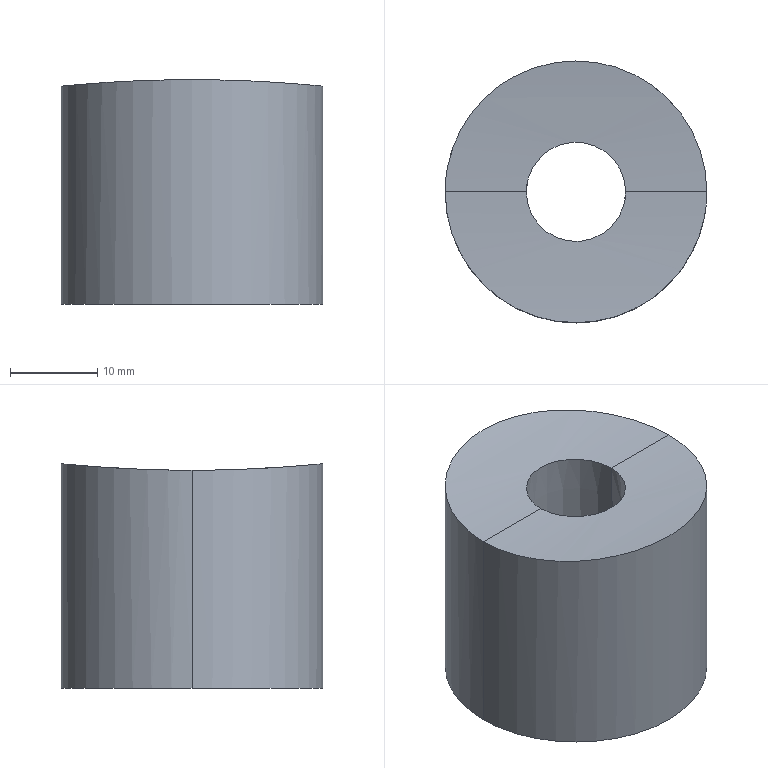Component | SolidWorks | JF21-80.1-1-3(_)-1-SOLID13-1 | 1 solid | 7 faces | box 30 x 30 x 25.75 mm | volume 14893 mm3 | cylinder 4 | cone 2 | plane 1 | commonest cylinder face diameters 300 x2 30 x2
STEP:
#1=COLOUR_RGB('',0.7922,0.8196,0.9333);
#2=FILL_AREA_STYLE_COLOUR('',#1);
#3=FILL_AREA_STYLE('',(#2));
#4=SURFACE_STYLE_FILL_AREA(#3);
#5=SURFACE_SIDE_STYLE('',(#4));
#6=SURFACE_STYLE_USAGE(.BOTH.,#5);
#7=PRESENTATION_STYLE_ASSIGNMENT((#6));
#8=CARTESIAN_POINT('',(10.8,-39.37,30.315));
#9=VERTEX_POINT('',#8);
#10=CARTESIAN_POINT('',(11.248,-39.37,30.315));
#11=VERTEX_POINT('',#10);
#12=CARTESIAN_POINT('',(10.8,-39.37,30.315));
#13=CARTESIAN_POINT('',(10.8,-39.385,30.315));
#14=CARTESIAN_POINT('',(10.801,-39.399,30.315));
#15=CARTESIAN_POINT('',(10.805,-39.421,30.315));
#16=CARTESIAN_POINT('',(10.807,-39.428,30.315));
#17=CARTESIAN_POINT('',(10.811,-39.442,30.315));
#18=CARTESIAN_POINT('',(10.814,-39.449,30.315));
#19=CARTESIAN_POINT('',(10.822,-39.469,30.316));
#20=CARTESIAN_POINT('',(10.829,-39.482,30.316));
#21=CARTESIAN_POINT('',(10.845,-39.507,30.317));
#22=CARTESIAN_POINT('',(10.855,-39.518,30.317));
#23=CARTESIAN_POINT('',(10.876,-39.539,30.317));
#24=CARTESIAN_POINT('',(10.887,-39.548,30.318));
#25=CARTESIAN_POINT('',(10.905,-39.56,30.318));
#26=CARTESIAN_POINT('',(10.912,-39.564,30.318));
#27=CARTESIAN_POINT('',(10.924,-39.571,30.318));
#28=CARTESIAN_POINT('',(10.931,-39.574,30.318));
#29=CARTESIAN_POINT('',(10.951,-39.583,30.319));
#30=CARTESIAN_POINT('',(10.965,-39.587,30.319));
#31=CARTESIAN_POINT('',(10.994,-39.593,30.319));
#32=CARTESIAN_POINT('',(11.009,-39.594,30.319));
#33=CARTESIAN_POINT('',(11.038,-39.594,30.319));
#34=CARTESIAN_POINT('',(11.053,-39.593,30.319));
#35=CARTESIAN_POINT('',(11.082,-39.587,30.319));
#36=CARTESIAN_POINT('',(11.096,-39.583,30.319));
#37=CARTESIAN_POINT('',(11.116,-39.574,30.318));
#38=CARTESIAN_POINT('',(11.123,-39.571,30.318));
#39=CARTESIAN_POINT('',(11.136,-39.564,30.318));
#40=CARTESIAN_POINT('',(11.142,-39.56,30.318));
#41=CARTESIAN_POINT('',(11.16,-39.548,30.318));
#42=CARTESIAN_POINT('',(11.171,-39.539,30.317));
#43=CARTESIAN_POINT('',(11.192,-39.518,30.317));
#44=CARTESIAN_POINT('',(11.202,-39.507,30.317));
#45=CARTESIAN_POINT('',(11.214,-39.489,30.316));
#46=CARTESIAN_POINT('',(11.218,-39.482,30.316));
#47=CARTESIAN_POINT('',(11.225,-39.469,30.316));
#48=CARTESIAN_POINT('',(11.228,-39.463,30.316));
#49=CARTESIAN_POINT('',(11.236,-39.442,30.315));
#50=CARTESIAN_POINT('',(11.24,-39.428,30.315));
#51=CARTESIAN_POINT('',(11.246,-39.4,30.315));
#52=CARTESIAN_POINT('',(11.248,-39.385,30.315));
#53=CARTESIAN_POINT('',(11.248,-39.37,30.315));
#54=B_SPLINE_CURVE_WITH_KNOTS('',3,(#12,#13,#14,#15,#16,#17,#18,#19,#20,#21,#22,#23,#24,#25,#26,#27,#28,#29,#30,#31,#32,#33,#34,#35,#36,#37,#38,#39,#40,#41,#42,#43,#44,#45,#46,#47,#48,#49,#50,#51,#52,#53),.UNSPECIFIED.,.F.,.F.,(4,2,2,2,2,2,2,2,2,2,2,2,2,2,2,2,2,2,2,2,4),(0.,0.001112,0.001667,0.002223,0.003335,0.004447,0.005558,0.006114,0.00667,0.007782,0.008893,0.01,0.01112,0.01167,0.01223,0.01334,0.01445,0.01501,0.01556,0.01667,0.01779),.UNSPECIFIED.);
#55=EDGE_CURVE('',#9,#11,#54,.T.);
#56=ORIENTED_EDGE('',*,*,#55,.T.);
#57=CARTESIAN_POINT('',(11.278,-39.37,29.331));
#58=VERTEX_POINT('',#57);
#59=CARTESIAN_POINT('',(11.278,-39.37,29.331));
#60=DIRECTION('',(-0.0312,-0.,0.9995));
#61=VECTOR('',#60,39.37);
#62=LINE('',#59,#61);
#63=EDGE_CURVE('',#58,#11,#62,.T.);
#64=ORIENTED_EDGE('',*,*,#63,.F.);
#65=CARTESIAN_POINT('',(10.769,-39.37,29.331));
#66=VERTEX_POINT('',#65);
#67=CARTESIAN_POINT('',(11.024,-39.37,29.331));
#68=DIRECTION('',(0.,0.,-1.));
#69=DIRECTION('',(-1.,0.,0.));
#70=AXIS2_PLACEMENT_3D('',#67,#68,#69);
#71=CIRCLE('',#70,0.2548);
#72=EDGE_CURVE('',#58,#66,#71,.T.);
#73=ORIENTED_EDGE('',*,*,#72,.T.);
#74=CARTESIAN_POINT('',(10.769,-39.37,29.331));
#75=DIRECTION('',(0.0312,0.,0.9995));
#76=VECTOR('',#75,39.37);
#77=LINE('',#74,#76);
#78=EDGE_CURVE('',#66,#9,#77,.T.);
#79=ORIENTED_EDGE('',*,*,#78,.T.);
#80=EDGE_LOOP('',(#56,#64,#73,#79));
#81=FACE_OUTER_BOUND('',#80,.T.);
#82=CARTESIAN_POINT('',(11.024,-39.37,29.331));
#83=DIRECTION('',(0.,0.,-1.));
#84=DIRECTION('',(1.,0.,0.));
#85=AXIS2_PLACEMENT_3D('',#82,#83,#84);
#86=CONICAL_SURFACE('',#85,0.2548,0.03121);
#87=ADVANCED_FACE('',(#81),#86,.F.);
#88=CARTESIAN_POINT('',(11.614,-39.37,30.315));
#89=VERTEX_POINT('',#88);
#90=CARTESIAN_POINT('',(10.433,-39.37,30.315));
#91=VERTEX_POINT('',#90);
#92=CARTESIAN_POINT('',(11.614,-39.37,30.315));
#93=CARTESIAN_POINT('',(11.614,-39.331,30.315));
#94=CARTESIAN_POINT('',(11.61,-39.293,30.315));
#95=CARTESIAN_POINT('',(11.599,-39.236,30.316));
#96=CARTESIAN_POINT('',(11.594,-39.217,30.317));
#97=CARTESIAN_POINT('',(11.583,-39.18,30.318));
#98=CARTESIAN_POINT('',(11.577,-39.162,30.319));
#99=CARTESIAN_POINT('',(11.554,-39.108,30.321));
#100=CARTESIAN_POINT('',(11.536,-39.074,30.322));
#101=CARTESIAN_POINT('',(11.504,-39.026,30.325));
#102=CARTESIAN_POINT('',(11.492,-39.01,30.326));
#103=CARTESIAN_POINT('',(11.468,-38.98,30.328));
#104=CARTESIAN_POINT('',(11.455,-38.966,30.329));
#105=CARTESIAN_POINT('',(11.414,-38.925,30.332));
#106=CARTESIAN_POINT('',(11.384,-38.901,30.334));
#107=CARTESIAN_POINT('',(11.336,-38.868,30.336));
#108=CARTESIAN_POINT('',(11.319,-38.858,30.337));
#109=CARTESIAN_POINT('',(11.285,-38.84,30.339));
#110=CARTESIAN_POINT('',(11.25,-38.824,30.34));
#111=CARTESIAN_POINT('',(11.214,-38.811,30.342));
#112=CARTESIAN_POINT('',(11.177,-38.799,30.343));
#113=CARTESIAN_POINT('',(11.158,-38.795,30.343));
#114=CARTESIAN_POINT('',(11.101,-38.783,30.344));
#115=CARTESIAN_POINT('',(11.063,-38.78,30.345));
#116=CARTESIAN_POINT('',(11.005,-38.78,30.345));
#117=CARTESIAN_POINT('',(10.985,-38.78,30.344));
#118=CARTESIAN_POINT('',(10.947,-38.784,30.344));
#119=CARTESIAN_POINT('',(10.927,-38.787,30.344));
#120=CARTESIAN_POINT('',(10.871,-38.798,30.343));
#121=CARTESIAN_POINT('',(10.834,-38.81,30.342));
#122=CARTESIAN_POINT('',(10.78,-38.832,30.34));
#123=CARTESIAN_POINT('',(10.762,-38.84,30.339));
#124=CARTESIAN_POINT('',(10.728,-38.858,30.337));
#125=CARTESIAN_POINT('',(10.712,-38.868,30.336));
#126=CARTESIAN_POINT('',(10.664,-38.9,30.334));
#127=CARTESIAN_POINT('',(10.634,-38.925,30.332));
#128=CARTESIAN_POINT('',(10.579,-38.98,30.328));
#129=CARTESIAN_POINT('',(10.554,-39.01,30.326));
#130=CARTESIAN_POINT('',(10.522,-39.057,30.323));
#131=CARTESIAN_POINT('',(10.512,-39.074,30.322));
#132=CARTESIAN_POINT('',(10.494,-39.108,30.321));
#133=CARTESIAN_POINT('',(10.486,-39.126,30.32));
#134=CARTESIAN_POINT('',(10.463,-39.179,30.318));
#135=CARTESIAN_POINT('',(10.452,-39.216,30.317));
#136=CARTESIAN_POINT('',(10.437,-39.292,30.315));
#137=CARTESIAN_POINT('',(10.433,-39.331,30.315));
#138=CARTESIAN_POINT('',(10.433,-39.37,30.315));
#139=B_SPLINE_CURVE_WITH_KNOTS('',3,(#92,#93,#94,#95,#96,#97,#98,#99,#100,#101,#102,#103,#104,#105,#106,#107,#108,#109,#110,#111,#112,#113,#114,#115,#116,#117,#118,#119,#120,#121,#122,#123,#124,#125,#126,#127,#128,#129,#130,#131,#132,#133,#134,#135,#136,#137,#138),.UNSPECIFIED.,.F.,.F.,(4,2,2,2,2,2,2,2,2,1,2,2,2,2,2,2,2,2,2,2,2,2,2,4),(0.,0.002932,0.004398,0.005864,0.008797,0.01026,0.01173,0.01466,0.01613,0.01759,0.01906,0.02053,0.02346,0.02492,0.02639,0.02932,0.03079,0.03225,0.03519,0.03812,0.03959,0.04105,0.04398,0.04692),.UNSPECIFIED.);
#140=EDGE_CURVE('',#89,#91,#139,.T.);
#141=ORIENTED_EDGE('',*,*,#140,.T.);
#142=CARTESIAN_POINT('',(-15.748,-39.37,30.315));
#143=DIRECTION('',(1.,0.,0.));
#144=VECTOR('',#143,39.37);
#145=LINE('',#142,#144);
#146=EDGE_CURVE('',#91,#9,#145,.T.);
#147=ORIENTED_EDGE('',*,*,#146,.T.);
#148=CARTESIAN_POINT('',(11.248,-39.37,30.315));
#149=CARTESIAN_POINT('',(11.248,-39.355,30.315));
#150=CARTESIAN_POINT('',(11.246,-39.341,30.315));
#151=CARTESIAN_POINT('',(11.242,-39.319,30.315));
#152=CARTESIAN_POINT('',(11.24,-39.312,30.315));
#153=CARTESIAN_POINT('',(11.236,-39.298,30.315));
#154=CARTESIAN_POINT('',(11.233,-39.291,30.315));
#155=CARTESIAN_POINT('',(11.225,-39.271,30.316));
#156=CARTESIAN_POINT('',(11.218,-39.258,30.316));
#157=CARTESIAN_POINT('',(11.202,-39.234,30.317));
#158=CARTESIAN_POINT('',(11.192,-39.222,30.317));
#159=CARTESIAN_POINT('',(11.172,-39.201,30.317));
#160=CARTESIAN_POINT('',(11.16,-39.192,30.318));
#161=CARTESIAN_POINT('',(11.142,-39.18,30.318));
#162=CARTESIAN_POINT('',(11.136,-39.176,30.318));
#163=CARTESIAN_POINT('',(11.123,-39.169,30.318));
#164=CARTESIAN_POINT('',(11.116,-39.166,30.318));
#165=CARTESIAN_POINT('',(11.096,-39.158,30.319));
#166=CARTESIAN_POINT('',(11.082,-39.153,30.319));
#167=CARTESIAN_POINT('',(11.053,-39.148,30.319));
#168=CARTESIAN_POINT('',(11.038,-39.146,30.319));
#169=CARTESIAN_POINT('',(11.009,-39.146,30.319));
#170=CARTESIAN_POINT('',(10.994,-39.148,30.319));
#171=CARTESIAN_POINT('',(10.966,-39.153,30.319));
#172=CARTESIAN_POINT('',(10.952,-39.158,30.319));
#173=CARTESIAN_POINT('',(10.931,-39.166,30.318));
#174=CARTESIAN_POINT('',(10.925,-39.169,30.318));
#175=CARTESIAN_POINT('',(10.912,-39.176,30.318));
#176=CARTESIAN_POINT('',(10.905,-39.18,30.318));
#177=CARTESIAN_POINT('',(10.887,-39.192,30.318));
#178=CARTESIAN_POINT('',(10.876,-39.201,30.317));
#179=CARTESIAN_POINT('',(10.855,-39.222,30.317));
#180=CARTESIAN_POINT('',(10.846,-39.233,30.317));
#181=CARTESIAN_POINT('',(10.833,-39.252,30.316));
#182=CARTESIAN_POINT('',(10.83,-39.258,30.316));
#183=CARTESIAN_POINT('',(10.823,-39.271,30.316));
#184=CARTESIAN_POINT('',(10.819,-39.277,30.316));
#185=CARTESIAN_POINT('',(10.811,-39.298,30.315));
#186=CARTESIAN_POINT('',(10.807,-39.312,30.315));
#187=CARTESIAN_POINT('',(10.801,-39.34,30.315));
#188=CARTESIAN_POINT('',(10.8,-39.355,30.315));
#189=CARTESIAN_POINT('',(10.8,-39.37,30.315));
#190=B_SPLINE_CURVE_WITH_KNOTS('',3,(#148,#149,#150,#151,#152,#153,#154,#155,#156,#157,#158,#159,#160,#161,#162,#163,#164,#165,#166,#167,#168,#169,#170,#171,#172,#173,#174,#175,#176,#177,#178,#179,#180,#181,#182,#183,#184,#185,#186,#187,#188,#189),.UNSPECIFIED.,.F.,.F.,(4,2,2,2,2,2,2,2,2,2,2,2,2,2,2,2,2,2,2,2,4),(0.,0.001112,0.001667,0.002223,0.003335,0.004447,0.005558,0.006114,0.00667,0.007782,0.008893,0.01,0.01112,0.01167,0.01223,0.01334,0.01445,0.01501,0.01556,0.01667,0.01779),.UNSPECIFIED.);
#191=EDGE_CURVE('',#11,#9,#190,.T.);
#192=ORIENTED_EDGE('',*,*,#191,.F.);
#193=CARTESIAN_POINT('',(-15.748,-39.37,30.315));
#194=DIRECTION('',(1.,0.,0.));
#195=VECTOR('',#194,39.37);
#196=LINE('',#193,#195);
#197=EDGE_CURVE('',#11,#89,#196,.T.);
#198=ORIENTED_EDGE('',*,*,#197,.T.);
#199=EDGE_LOOP('',(#141,#147,#192,#198));
#200=FACE_OUTER_BOUND('',#199,.T.);
#201=CARTESIAN_POINT('',(-15.748,-39.37,36.22));
#202=DIRECTION('',(1.,0.,0.));
#203=DIRECTION('',(0.,0.,1.));
#204=AXIS2_PLACEMENT_3D('',#201,#202,#203);
#205=CYLINDRICAL_SURFACE('',#204,5.906);
#206=ADVANCED_FACE('',(#200),#205,.F.);
#207=ORIENTED_EDGE('',*,*,#140,.F.);
#208=CARTESIAN_POINT('',(11.614,-39.37,29.331));
#209=VERTEX_POINT('',#208);
#210=CARTESIAN_POINT('',(11.614,-39.37,30.709));
#211=DIRECTION('',(0.,0.,1.));
#212=VECTOR('',#211,39.37);
#213=LINE('',#210,#212);
#214=EDGE_CURVE('',#209,#89,#213,.T.);
#215=ORIENTED_EDGE('',*,*,#214,.F.);
#216=CARTESIAN_POINT('',(10.433,-39.37,29.331));
#217=VERTEX_POINT('',#216);
#218=CARTESIAN_POINT('',(11.024,-39.37,29.331));
#219=DIRECTION('',(0.,0.,1.));
#220=DIRECTION('',(1.,0.,0.));
#221=AXIS2_PLACEMENT_3D('',#218,#219,#220);
#222=CIRCLE('',#221,0.5906);
#223=EDGE_CURVE('',#209,#217,#222,.T.);
#224=ORIENTED_EDGE('',*,*,#223,.T.);
#225=CARTESIAN_POINT('',(10.433,-39.37,30.709));
#226=DIRECTION('',(0.,0.,1.));
#227=VECTOR('',#226,39.37);
#228=LINE('',#225,#227);
#229=EDGE_CURVE('',#217,#91,#228,.T.);
#230=ORIENTED_EDGE('',*,*,#229,.T.);
#231=EDGE_LOOP('',(#207,#215,#224,#230));
#232=FACE_OUTER_BOUND('',#231,.T.);
#233=CARTESIAN_POINT('',(11.024,-39.37,30.709));
#234=DIRECTION('',(0.,0.,-1.));
#235=DIRECTION('',(1.,0.,0.));
#236=AXIS2_PLACEMENT_3D('',#233,#234,#235);
#237=CYLINDRICAL_SURFACE('',#236,0.5906);
#238=ADVANCED_FACE('',(#232),#237,.T.);
#239=ORIENTED_EDGE('',*,*,#214,.T.);
#240=CARTESIAN_POINT('',(10.433,-39.37,30.315));
#241=CARTESIAN_POINT('',(10.433,-39.409,30.315));
#242=CARTESIAN_POINT('',(10.437,-39.447,30.315));
#243=CARTESIAN_POINT('',(10.448,-39.504,30.316));
#244=CARTESIAN_POINT('',(10.453,-39.523,30.317));
#245=CARTESIAN_POINT('',(10.464,-39.56,30.318));
#246=CARTESIAN_POINT('',(10.471,-39.578,30.319));
#247=CARTESIAN_POINT('',(10.493,-39.632,30.321));
#248=CARTESIAN_POINT('',(10.511,-39.666,30.322));
#249=CARTESIAN_POINT('',(10.543,-39.714,30.325));
#250=CARTESIAN_POINT('',(10.555,-39.73,30.326));
#251=CARTESIAN_POINT('',(10.579,-39.76,30.328));
#252=CARTESIAN_POINT('',(10.592,-39.774,30.329));
#253=CARTESIAN_POINT('',(10.633,-39.815,30.332));
#254=CARTESIAN_POINT('',(10.663,-39.839,30.334));
#255=CARTESIAN_POINT('',(10.711,-39.872,30.336));
#256=CARTESIAN_POINT('',(10.728,-39.882,30.337));
#257=CARTESIAN_POINT('',(10.762,-39.9,30.339));
#258=CARTESIAN_POINT('',(10.797,-39.916,30.34));
#259=CARTESIAN_POINT('',(10.833,-39.929,30.342));
#260=CARTESIAN_POINT('',(10.87,-39.941,30.343));
#261=CARTESIAN_POINT('',(10.889,-39.945,30.343));
#262=CARTESIAN_POINT('',(10.946,-39.957,30.344));
#263=CARTESIAN_POINT('',(10.985,-39.961,30.345));
#264=CARTESIAN_POINT('',(11.042,-39.961,30.345));
#265=CARTESIAN_POINT('',(11.062,-39.96,30.344));
#266=CARTESIAN_POINT('',(11.101,-39.956,30.344));
#267=CARTESIAN_POINT('',(11.12,-39.953,30.344));
#268=CARTESIAN_POINT('',(11.177,-39.942,30.343));
#269=CARTESIAN_POINT('',(11.213,-39.931,30.342));
#270=CARTESIAN_POINT('',(11.267,-39.908,30.34));
#271=CARTESIAN_POINT('',(11.285,-39.9,30.339));
#272=CARTESIAN_POINT('',(11.319,-39.882,30.337));
#273=CARTESIAN_POINT('',(11.336,-39.872,30.336));
#274=CARTESIAN_POINT('',(11.384,-39.84,30.334));
#275=CARTESIAN_POINT('',(11.413,-39.815,30.332));
#276=CARTESIAN_POINT('',(11.469,-39.76,30.328));
#277=CARTESIAN_POINT('',(11.493,-39.731,30.326));
#278=CARTESIAN_POINT('',(11.525,-39.683,30.323));
#279=CARTESIAN_POINT('',(11.535,-39.666,30.322));
#280=CARTESIAN_POINT('',(11.553,-39.632,30.321));
#281=CARTESIAN_POINT('',(11.562,-39.614,30.32));
#282=CARTESIAN_POINT('',(11.584,-39.561,30.318));
#283=CARTESIAN_POINT('',(11.595,-39.524,30.317));
#284=CARTESIAN_POINT('',(11.61,-39.448,30.315));
#285=CARTESIAN_POINT('',(11.614,-39.409,30.315));
#286=CARTESIAN_POINT('',(11.614,-39.37,30.315));
#287=B_SPLINE_CURVE_WITH_KNOTS('',3,(#240,#241,#242,#243,#244,#245,#246,#247,#248,#249,#250,#251,#252,#253,#254,#255,#256,#257,#258,#259,#260,#261,#262,#263,#264,#265,#266,#267,#268,#269,#270,#271,#272,#273,#274,#275,#276,#277,#278,#279,#280,#281,#282,#283,#284,#285,#286),.UNSPECIFIED.,.F.,.F.,(4,2,2,2,2,2,2,2,2,1,2,2,2,2,2,2,2,2,2,2,2,2,2,4),(0.,0.002932,0.004398,0.005864,0.008797,0.01026,0.01173,0.01466,0.01613,0.01759,0.01906,0.02053,0.02346,0.02492,0.02639,0.02932,0.03079,0.03225,0.03519,0.03812,0.03959,0.04105,0.04398,0.04692),.UNSPECIFIED.);
#288=EDGE_CURVE('',#91,#89,#287,.T.);
#289=ORIENTED_EDGE('',*,*,#288,.F.);
#290=ORIENTED_EDGE('',*,*,#229,.F.);
#291=CARTESIAN_POINT('',(11.024,-39.37,29.331));
#292=DIRECTION('',(0.,0.,1.));
#293=DIRECTION('',(1.,0.,0.));
#294=AXIS2_PLACEMENT_3D('',#291,#292,#293);
#295=CIRCLE('',#294,0.5906);
#296=EDGE_CURVE('',#217,#209,#295,.T.);
#297=ORIENTED_EDGE('',*,*,#296,.T.);
#298=EDGE_LOOP('',(#239,#289,#290,#297));
#299=FACE_OUTER_BOUND('',#298,.T.);
#300=CARTESIAN_POINT('',(11.024,-39.37,30.709));
#301=DIRECTION('',(0.,0.,-1.));
#302=DIRECTION('',(1.,0.,0.));
#303=AXIS2_PLACEMENT_3D('',#300,#301,#302);
#304=CYLINDRICAL_SURFACE('',#303,0.5906);
#305=ADVANCED_FACE('',(#299),#304,.T.);
#306=CARTESIAN_POINT('',(11.024,-39.37,29.331));
#307=DIRECTION('',(0.,0.,-1.));
#308=DIRECTION('',(-1.,0.,0.));
#309=AXIS2_PLACEMENT_3D('',#306,#307,#308);
#310=CIRCLE('',#309,0.2548);
#311=EDGE_CURVE('',#66,#58,#310,.T.);
#312=ORIENTED_EDGE('',*,*,#311,.F.);
#313=ORIENTED_EDGE('',*,*,#72,.F.);
#314=EDGE_LOOP('',(#312,#313));
#315=FACE_BOUND('',#314,.T.);
#316=ORIENTED_EDGE('',*,*,#296,.F.);
#317=ORIENTED_EDGE('',*,*,#223,.F.);
#318=EDGE_LOOP('',(#316,#317));
#319=FACE_OUTER_BOUND('',#318,.T.);
#320=CARTESIAN_POINT('',(11.024,-39.37,29.331));
#321=DIRECTION('',(0.,0.,1.));
#322=DIRECTION('',(-1.,0.,0.));
#323=AXIS2_PLACEMENT_3D('',#320,#321,#322);
#324=PLANE('',#323);
#325=ADVANCED_FACE('',(#315,#319),#324,.F.);
#326=ORIENTED_EDGE('',*,*,#146,.F.);
#327=ORIENTED_EDGE('',*,*,#288,.T.);
#328=ORIENTED_EDGE('',*,*,#197,.F.);
#329=ORIENTED_EDGE('',*,*,#55,.F.);
#330=EDGE_LOOP('',(#326,#327,#328,#329));
#331=FACE_OUTER_BOUND('',#330,.T.);
#332=CARTESIAN_POINT('',(-15.748,-39.37,36.22));
#333=DIRECTION('',(1.,0.,0.));
#334=DIRECTION('',(0.,0.,1.));
#335=AXIS2_PLACEMENT_3D('',#332,#333,#334);
#336=CYLINDRICAL_SURFACE('',#335,5.906);
#337=ADVANCED_FACE('',(#331),#336,.F.);
#338=ORIENTED_EDGE('',*,*,#63,.T.);
#339=ORIENTED_EDGE('',*,*,#191,.T.);
#340=ORIENTED_EDGE('',*,*,#78,.F.);
#341=ORIENTED_EDGE('',*,*,#311,.T.);
#342=EDGE_LOOP('',(#338,#339,#340,#341));
#343=FACE_OUTER_BOUND('',#342,.T.);
#344=CARTESIAN_POINT('',(11.024,-39.37,29.331));
#345=DIRECTION('',(0.,0.,-1.));
#346=DIRECTION('',(1.,0.,0.));
#347=AXIS2_PLACEMENT_3D('',#344,#345,#346);
#348=CONICAL_SURFACE('',#347,0.2548,0.03121);
#349=ADVANCED_FACE('',(#343),#348,.F.);
#350=CLOSED_SHELL('',(#87,#206,#238,#305,#325,#337,#349));
#351=MANIFOLD_SOLID_BREP('',#350);
#352=STYLED_ITEM('',(#7),#351);
#353=(LENGTH_UNIT()NAMED_UNIT(*)SI_UNIT($,.METRE.));
#354=LENGTH_MEASURE_WITH_UNIT(LENGTH_MEASURE(0.0254),#353);
#355=DIMENSIONAL_EXPONENTS(1.,0.,0.,0.,0.,0.,0.);
#356=(CONVERSION_BASED_UNIT('',#354)LENGTH_UNIT()NAMED_UNIT(#355));
#357=UNCERTAINTY_MEASURE_WITH_UNIT(LENGTH_MEASURE(0.00001),#356,'','');
#358=(NAMED_UNIT(*)PLANE_ANGLE_UNIT()SI_UNIT($,.RADIAN.));
#359=(NAMED_UNIT(*)SI_UNIT($,.STERADIAN.)SOLID_ANGLE_UNIT());
#360=(GEOMETRIC_REPRESENTATION_CONTEXT(3)GLOBAL_UNCERTAINTY_ASSIGNED_CONTEXT((#357))GLOBAL_UNIT_ASSIGNED_CONTEXT((#356,#358,#359))REPRESENTATION_CONTEXT('',''));
#361=MECHANICAL_DESIGN_GEOMETRIC_PRESENTATION_REPRESENTATION('',(#352),#360);
#362=CARTESIAN_POINT('',(0.,0.,0.));
#363=DIRECTION('',(0.,0.,1.));
#364=DIRECTION('',(1.,0.,0.));
#365=AXIS2_PLACEMENT_3D('',#362,#363,#364);
#366=(LENGTH_UNIT()NAMED_UNIT(*)SI_UNIT($,.METRE.));
#367=LENGTH_MEASURE_WITH_UNIT(LENGTH_MEASURE(0.0254),#366);
#368=DIMENSIONAL_EXPONENTS(1.,0.,0.,0.,0.,0.,0.);
#369=(CONVERSION_BASED_UNIT('',#367)LENGTH_UNIT()NAMED_UNIT(#368));
#370=UNCERTAINTY_MEASURE_WITH_UNIT(LENGTH_MEASURE(0.00001),#369,'','');
#371=(NAMED_UNIT(*)PLANE_ANGLE_UNIT()SI_UNIT($,.RADIAN.));
#372=(NAMED_UNIT(*)SI_UNIT($,.STERADIAN.)SOLID_ANGLE_UNIT());
#373=(GEOMETRIC_REPRESENTATION_CONTEXT(3)GLOBAL_UNCERTAINTY_ASSIGNED_CONTEXT((#370))GLOBAL_UNIT_ASSIGNED_CONTEXT((#369,#371,#372))REPRESENTATION_CONTEXT('',''));
#374=ADVANCED_BREP_SHAPE_REPRESENTATION('',(#351,#365),#373);
#375=PRESENTATION_LAYER_ASSIGNMENT('','',(#352));